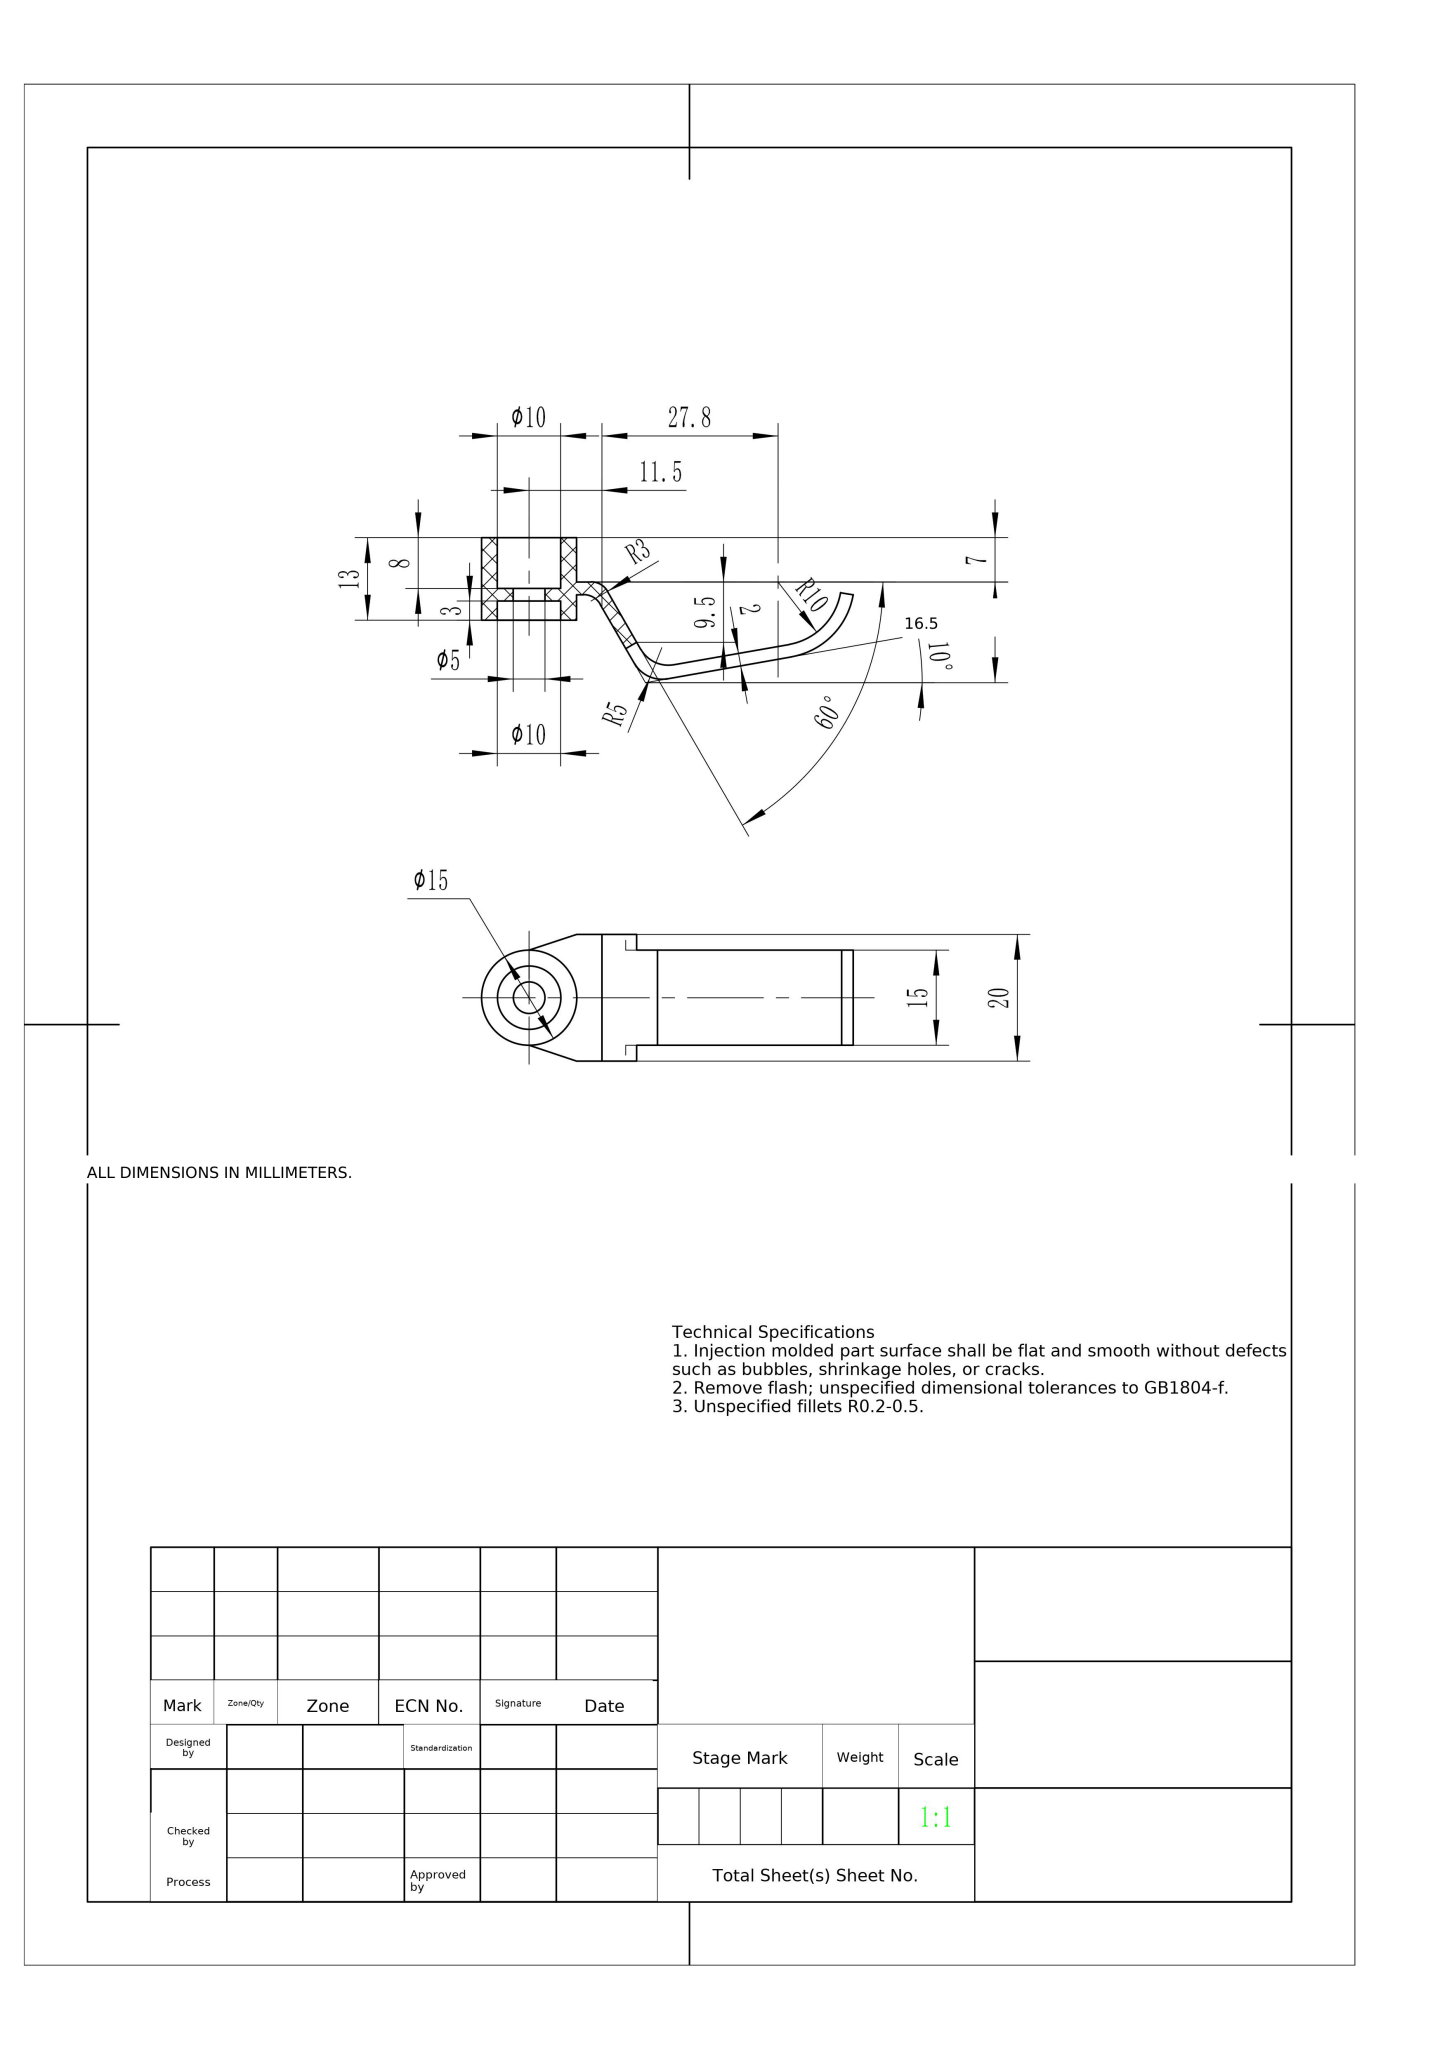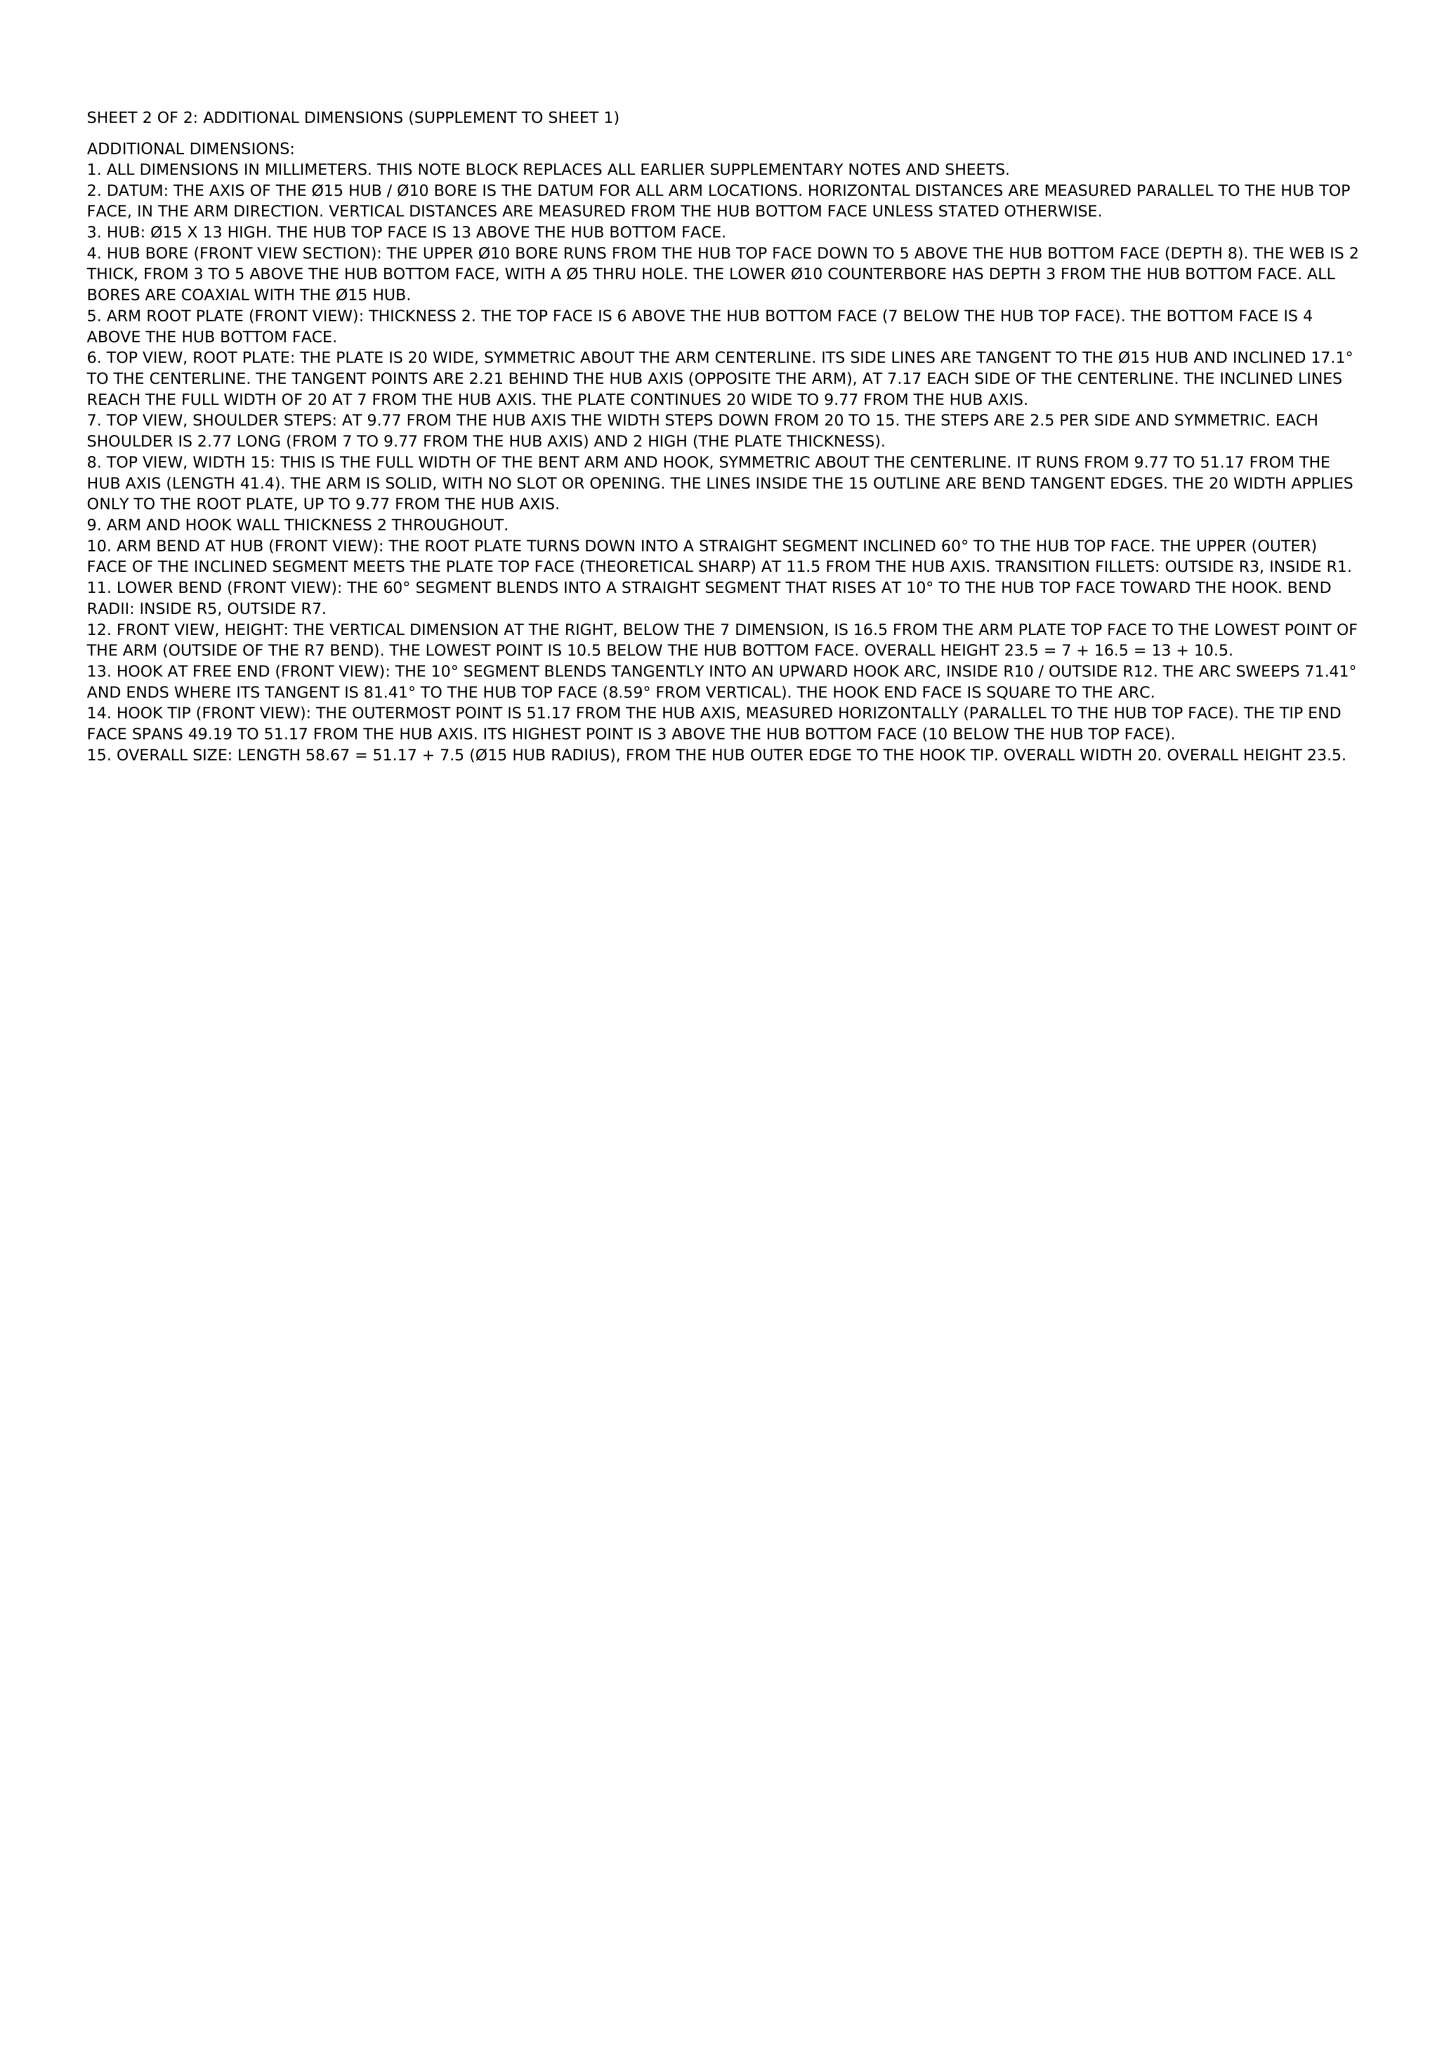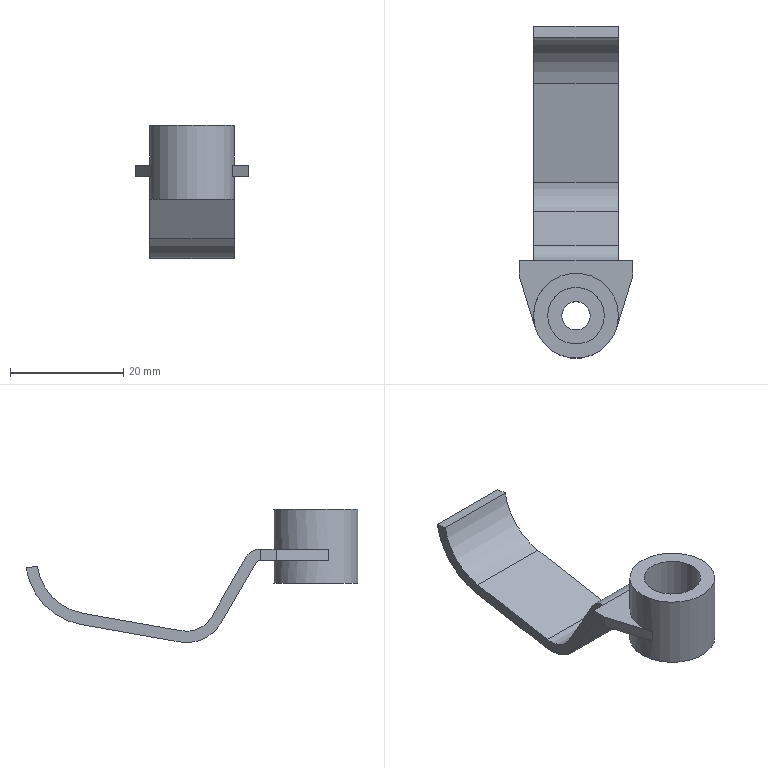Part | NX | mm | 1 solid | 29 faces | box 20 x 58.67 x 23.5 mm | volume 3167 mm3 | plane 19 | cylinder 10 | commonest cylinder face diameters 10 x3 2 x1 14 x1 24 x1 20 x1 6 x1 15 x1 5 x1
STEP:
#1=CARTESIAN_POINT('',(0.,0.,0.));
#2=DIRECTION('',(0.,0.,1.));
#3=DIRECTION('',(1.,0.,0.));
#4=AXIS2_PLACEMENT_3D('',#1,#2,#3);
#5=(LENGTH_UNIT()NAMED_UNIT(*)SI_UNIT(.MILLI.,.METRE.));
#6=UNCERTAINTY_MEASURE_WITH_UNIT(LENGTH_MEASURE(0.00002),#5,'','');
#7=(NAMED_UNIT(*)PLANE_ANGLE_UNIT()SI_UNIT($,.RADIAN.));
#8=PLANE_ANGLE_MEASURE_WITH_UNIT(PLANE_ANGLE_MEASURE(0.01745),#7);
#9=DIMENSIONAL_EXPONENTS(0.,0.,0.,0.,0.,0.,0.);
#10=(CONVERSION_BASED_UNIT('',#8)NAMED_UNIT(#9)PLANE_ANGLE_UNIT());
#11=(NAMED_UNIT(*)SI_UNIT($,.STERADIAN.)SOLID_ANGLE_UNIT());
#12=(GEOMETRIC_REPRESENTATION_CONTEXT(3)GLOBAL_UNCERTAINTY_ASSIGNED_CONTEXT((#6))GLOBAL_UNIT_ASSIGNED_CONTEXT((#5,#10,#11))REPRESENTATION_CONTEXT('',''));
#13=SHAPE_REPRESENTATION('',(#4),#12);
#14=CARTESIAN_POINT('',(10.,9.768,6.));
#15=VERTEX_POINT('',#14);
#16=CARTESIAN_POINT('',(10.,9.768,4.));
#17=VERTEX_POINT('',#16);
#18=CARTESIAN_POINT('',(10.,9.768,8.));
#19=DIRECTION('',(0.,0.,-1.));
#20=VECTOR('',#19,1.);
#21=LINE('',#18,#20);
#22=EDGE_CURVE('',#15,#17,#21,.T.);
#23=ORIENTED_EDGE('',*,*,#22,.F.);
#24=CARTESIAN_POINT('',(10.,7.,6.));
#25=VERTEX_POINT('',#24);
#26=CARTESIAN_POINT('',(10.,9.768,6.));
#27=DIRECTION('',(0.,-1.,-0.));
#28=VECTOR('',#27,1.);
#29=LINE('',#26,#28);
#30=EDGE_CURVE('',#15,#25,#29,.T.);
#31=ORIENTED_EDGE('',*,*,#30,.T.);
#32=CARTESIAN_POINT('',(10.,7.,4.));
#33=VERTEX_POINT('',#32);
#34=CARTESIAN_POINT('',(10.,7.,6.));
#35=DIRECTION('',(0.,0.,-1.));
#36=VECTOR('',#35,1.);
#37=LINE('',#34,#36);
#38=EDGE_CURVE('',#25,#33,#37,.T.);
#39=ORIENTED_EDGE('',*,*,#38,.T.);
#40=CARTESIAN_POINT('',(10.,7.,4.));
#41=DIRECTION('',(0.,1.,0.));
#42=VECTOR('',#41,1.);
#43=LINE('',#40,#42);
#44=EDGE_CURVE('',#33,#17,#43,.T.);
#45=ORIENTED_EDGE('',*,*,#44,.T.);
#46=EDGE_LOOP('',(#23,#31,#39,#45));
#47=FACE_OUTER_BOUND('',#46,.T.);
#48=CARTESIAN_POINT('',(10.,9.768,3.));
#49=DIRECTION('',(-1.,0.,0.));
#50=DIRECTION('',(0.,0.,1.));
#51=AXIS2_PLACEMENT_3D('',#48,#49,#50);
#52=PLANE('',#51);
#53=ADVANCED_FACE('',(#47),#52,.F.);
#54=CARTESIAN_POINT('',(7.5,10.634,3.5));
#55=VERTEX_POINT('',#54);
#56=CARTESIAN_POINT('',(-7.5,10.634,3.5));
#57=VERTEX_POINT('',#56);
#58=CARTESIAN_POINT('',(10.,10.634,3.5));
#59=DIRECTION('',(-1.,0.,0.));
#60=VECTOR('',#59,1.);
#61=LINE('',#58,#60);
#62=EDGE_CURVE('',#55,#57,#61,.T.);
#63=ORIENTED_EDGE('',*,*,#62,.F.);
#64=CARTESIAN_POINT('',(7.5,9.768,4.));
#65=VERTEX_POINT('',#64);
#66=CARTESIAN_POINT('',(7.5,9.768,3.));
#67=DIRECTION('',(1.,-0.,-0.));
#68=DIRECTION('',(0.,-1.,0.));
#69=AXIS2_PLACEMENT_3D('',#66,#67,#68);
#70=CIRCLE('',#69,1.);
#71=EDGE_CURVE('',#55,#65,#70,.T.);
#72=ORIENTED_EDGE('',*,*,#71,.T.);
#73=CARTESIAN_POINT('',(-7.5,9.768,4.));
#74=VERTEX_POINT('',#73);
#75=CARTESIAN_POINT('',(10.,9.768,4.));
#76=DIRECTION('',(-1.,0.,0.));
#77=VECTOR('',#76,1.);
#78=LINE('',#75,#77);
#79=EDGE_CURVE('',#65,#74,#78,.T.);
#80=ORIENTED_EDGE('',*,*,#79,.T.);
#81=CARTESIAN_POINT('',(-7.5,9.768,3.));
#82=DIRECTION('',(1.,0.,0.));
#83=DIRECTION('',(0.,-1.,0.));
#84=AXIS2_PLACEMENT_3D('',#81,#82,#83);
#85=CIRCLE('',#84,1.);
#86=EDGE_CURVE('',#57,#74,#85,.T.);
#87=ORIENTED_EDGE('',*,*,#86,.F.);
#88=EDGE_LOOP('',(#63,#72,#80,#87));
#89=FACE_OUTER_BOUND('',#88,.T.);
#90=CARTESIAN_POINT('',(10.,9.768,3.));
#91=DIRECTION('',(-1.,0.,0.));
#92=DIRECTION('',(0.,0.,1.));
#93=AXIS2_PLACEMENT_3D('',#90,#91,#92);
#94=CYLINDRICAL_SURFACE('',#93,1.);
#95=ADVANCED_FACE('',(#89),#94,.F.);
#96=CARTESIAN_POINT('',(7.5,16.696,-7.));
#97=VERTEX_POINT('',#96);
#98=CARTESIAN_POINT('',(-7.5,16.696,-7.));
#99=VERTEX_POINT('',#98);
#100=CARTESIAN_POINT('',(10.,16.696,-7.));
#101=DIRECTION('',(-1.,0.,0.));
#102=VECTOR('',#101,1.);
#103=LINE('',#100,#102);
#104=EDGE_CURVE('',#97,#99,#103,.T.);
#105=ORIENTED_EDGE('',*,*,#104,.F.);
#106=CARTESIAN_POINT('',(7.5,10.634,3.5));
#107=DIRECTION('',(-0.,-0.5,0.866));
#108=VECTOR('',#107,1.);
#109=LINE('',#106,#108);
#110=EDGE_CURVE('',#97,#55,#109,.T.);
#111=ORIENTED_EDGE('',*,*,#110,.T.);
#112=ORIENTED_EDGE('',*,*,#62,.T.);
#113=CARTESIAN_POINT('',(-7.5,10.634,3.5));
#114=DIRECTION('',(0.,-0.5,0.866));
#115=VECTOR('',#114,1.);
#116=LINE('',#113,#115);
#117=EDGE_CURVE('',#99,#57,#116,.T.);
#118=ORIENTED_EDGE('',*,*,#117,.F.);
#119=EDGE_LOOP('',(#105,#111,#112,#118));
#120=FACE_OUTER_BOUND('',#119,.T.);
#121=CARTESIAN_POINT('',(10.,10.634,3.5));
#122=DIRECTION('',(0.,0.866,0.5));
#123=DIRECTION('',(0.,-0.5,0.866));
#124=AXIS2_PLACEMENT_3D('',#121,#122,#123);
#125=PLANE('',#124);
#126=ADVANCED_FACE('',(#120),#125,.F.);
#127=CARTESIAN_POINT('',(7.5,23.974,-10.394));
#128=VERTEX_POINT('',#127);
#129=CARTESIAN_POINT('',(-7.5,23.974,-10.394));
#130=VERTEX_POINT('',#129);
#131=CARTESIAN_POINT('',(10.,23.974,-10.394));
#132=DIRECTION('',(-1.,0.,0.));
#133=VECTOR('',#132,1.);
#134=LINE('',#131,#133);
#135=EDGE_CURVE('',#128,#130,#134,.T.);
#136=ORIENTED_EDGE('',*,*,#135,.F.);
#137=CARTESIAN_POINT('',(7.5,22.758,-3.5));
#138=DIRECTION('',(-1.,0.,0.));
#139=DIRECTION('',(-0.,-1.,0.));
#140=AXIS2_PLACEMENT_3D('',#137,#138,#139);
#141=CIRCLE('',#140,7.);
#142=EDGE_CURVE('',#128,#97,#141,.T.);
#143=ORIENTED_EDGE('',*,*,#142,.T.);
#144=ORIENTED_EDGE('',*,*,#104,.T.);
#145=CARTESIAN_POINT('',(-7.5,22.758,-3.5));
#146=DIRECTION('',(-1.,-0.,-0.));
#147=DIRECTION('',(0.,-1.,0.));
#148=AXIS2_PLACEMENT_3D('',#145,#146,#147);
#149=CIRCLE('',#148,7.);
#150=EDGE_CURVE('',#130,#99,#149,.T.);
#151=ORIENTED_EDGE('',*,*,#150,.F.);
#152=EDGE_LOOP('',(#136,#143,#144,#151));
#153=FACE_OUTER_BOUND('',#152,.T.);
#154=CARTESIAN_POINT('',(10.,22.758,-3.5));
#155=DIRECTION('',(-1.,0.,0.));
#156=DIRECTION('',(0.,0.,1.));
#157=AXIS2_PLACEMENT_3D('',#154,#155,#156);
#158=CYLINDRICAL_SURFACE('',#157,7.);
#159=ADVANCED_FACE('',(#153),#158,.T.);
#160=CARTESIAN_POINT('',(7.5,41.384,-7.324));
#161=VERTEX_POINT('',#160);
#162=CARTESIAN_POINT('',(-7.5,41.384,-7.324));
#163=VERTEX_POINT('',#162);
#164=CARTESIAN_POINT('',(10.,41.384,-7.324));
#165=DIRECTION('',(-1.,0.,0.));
#166=VECTOR('',#165,1.);
#167=LINE('',#164,#166);
#168=EDGE_CURVE('',#161,#163,#167,.T.);
#169=ORIENTED_EDGE('',*,*,#168,.F.);
#170=CARTESIAN_POINT('',(7.5,23.974,-10.394));
#171=DIRECTION('',(-0.,-0.9848,-0.1736));
#172=VECTOR('',#171,1.);
#173=LINE('',#170,#172);
#174=EDGE_CURVE('',#161,#128,#173,.T.);
#175=ORIENTED_EDGE('',*,*,#174,.T.);
#176=ORIENTED_EDGE('',*,*,#135,.T.);
#177=CARTESIAN_POINT('',(-7.5,23.974,-10.394));
#178=DIRECTION('',(0.,-0.9848,-0.1736));
#179=VECTOR('',#178,1.);
#180=LINE('',#177,#179);
#181=EDGE_CURVE('',#163,#130,#180,.T.);
#182=ORIENTED_EDGE('',*,*,#181,.F.);
#183=EDGE_LOOP('',(#169,#175,#176,#182));
#184=FACE_OUTER_BOUND('',#183,.T.);
#185=CARTESIAN_POINT('',(10.,23.974,-10.394));
#186=DIRECTION('',(0.,-0.1736,0.9848));
#187=DIRECTION('',(0.,-0.9848,-0.1736));
#188=AXIS2_PLACEMENT_3D('',#185,#186,#187);
#189=PLANE('',#188);
#190=ADVANCED_FACE('',(#184),#189,.F.);
#191=CARTESIAN_POINT('',(7.5,51.165,2.701));
#192=VERTEX_POINT('',#191);
#193=CARTESIAN_POINT('',(-7.5,51.165,2.701));
#194=VERTEX_POINT('',#193);
#195=CARTESIAN_POINT('',(10.,51.165,2.701));
#196=DIRECTION('',(-1.,0.,0.));
#197=VECTOR('',#196,1.);
#198=LINE('',#195,#197);
#199=EDGE_CURVE('',#192,#194,#198,.T.);
#200=ORIENTED_EDGE('',*,*,#199,.F.);
#201=CARTESIAN_POINT('',(7.5,39.3,4.494));
#202=DIRECTION('',(-1.,0.,0.));
#203=DIRECTION('',(-0.,-1.,0.));
#204=AXIS2_PLACEMENT_3D('',#201,#202,#203);
#205=CIRCLE('',#204,12.);
#206=EDGE_CURVE('',#192,#161,#205,.T.);
#207=ORIENTED_EDGE('',*,*,#206,.T.);
#208=ORIENTED_EDGE('',*,*,#168,.T.);
#209=CARTESIAN_POINT('',(-7.5,39.3,4.494));
#210=DIRECTION('',(-1.,-0.,-0.));
#211=DIRECTION('',(0.,-1.,0.));
#212=AXIS2_PLACEMENT_3D('',#209,#210,#211);
#213=CIRCLE('',#212,12.);
#214=EDGE_CURVE('',#194,#163,#213,.T.);
#215=ORIENTED_EDGE('',*,*,#214,.F.);
#216=EDGE_LOOP('',(#200,#207,#208,#215));
#217=FACE_OUTER_BOUND('',#216,.T.);
#218=CARTESIAN_POINT('',(10.,39.3,4.494));
#219=DIRECTION('',(-1.,0.,0.));
#220=DIRECTION('',(0.,0.,1.));
#221=AXIS2_PLACEMENT_3D('',#218,#219,#220);
#222=CYLINDRICAL_SURFACE('',#221,12.);
#223=ADVANCED_FACE('',(#217),#222,.T.);
#224=CARTESIAN_POINT('',(7.5,49.188,3.));
#225=VERTEX_POINT('',#224);
#226=CARTESIAN_POINT('',(-7.5,49.188,3.));
#227=VERTEX_POINT('',#226);
#228=CARTESIAN_POINT('',(10.,49.188,3.));
#229=DIRECTION('',(-1.,0.,0.));
#230=VECTOR('',#229,1.);
#231=LINE('',#228,#230);
#232=EDGE_CURVE('',#225,#227,#231,.T.);
#233=ORIENTED_EDGE('',*,*,#232,.F.);
#234=CARTESIAN_POINT('',(7.5,51.165,2.701));
#235=DIRECTION('',(0.,0.9888,-0.1494));
#236=VECTOR('',#235,1.);
#237=LINE('',#234,#236);
#238=EDGE_CURVE('',#225,#192,#237,.T.);
#239=ORIENTED_EDGE('',*,*,#238,.T.);
#240=ORIENTED_EDGE('',*,*,#199,.T.);
#241=CARTESIAN_POINT('',(-7.5,51.165,2.701));
#242=DIRECTION('',(-0.,0.9888,-0.1494));
#243=VECTOR('',#242,1.);
#244=LINE('',#241,#243);
#245=EDGE_CURVE('',#227,#194,#244,.T.);
#246=ORIENTED_EDGE('',*,*,#245,.F.);
#247=EDGE_LOOP('',(#233,#239,#240,#246));
#248=FACE_OUTER_BOUND('',#247,.T.);
#249=CARTESIAN_POINT('',(10.,51.165,2.701));
#250=DIRECTION('',(0.,-0.1494,-0.9888));
#251=DIRECTION('',(0.,0.9888,-0.1494));
#252=AXIS2_PLACEMENT_3D('',#249,#250,#251);
#253=PLANE('',#252);
#254=ADVANCED_FACE('',(#248),#253,.F.);
#255=CARTESIAN_POINT('',(7.5,41.036,-5.354));
#256=VERTEX_POINT('',#255);
#257=CARTESIAN_POINT('',(-7.5,41.036,-5.354));
#258=VERTEX_POINT('',#257);
#259=CARTESIAN_POINT('',(10.,41.036,-5.354));
#260=DIRECTION('',(-1.,0.,0.));
#261=VECTOR('',#260,1.);
#262=LINE('',#259,#261);
#263=EDGE_CURVE('',#256,#258,#262,.T.);
#264=ORIENTED_EDGE('',*,*,#263,.F.);
#265=CARTESIAN_POINT('',(7.5,39.3,4.494));
#266=DIRECTION('',(1.,-0.,-0.));
#267=DIRECTION('',(-0.,-1.,0.));
#268=AXIS2_PLACEMENT_3D('',#265,#266,#267);
#269=CIRCLE('',#268,10.);
#270=EDGE_CURVE('',#256,#225,#269,.T.);
#271=ORIENTED_EDGE('',*,*,#270,.T.);
#272=ORIENTED_EDGE('',*,*,#232,.T.);
#273=CARTESIAN_POINT('',(-7.5,39.3,4.494));
#274=DIRECTION('',(1.,0.,0.));
#275=DIRECTION('',(0.,-1.,0.));
#276=AXIS2_PLACEMENT_3D('',#273,#274,#275);
#277=CIRCLE('',#276,10.);
#278=EDGE_CURVE('',#258,#227,#277,.T.);
#279=ORIENTED_EDGE('',*,*,#278,.F.);
#280=EDGE_LOOP('',(#264,#271,#272,#279));
#281=FACE_OUTER_BOUND('',#280,.T.);
#282=CARTESIAN_POINT('',(10.,39.3,4.494));
#283=DIRECTION('',(-1.,0.,0.));
#284=DIRECTION('',(0.,0.,1.));
#285=AXIS2_PLACEMENT_3D('',#282,#283,#284);
#286=CYLINDRICAL_SURFACE('',#285,10.);
#287=ADVANCED_FACE('',(#281),#286,.F.);
#288=CARTESIAN_POINT('',(7.5,23.627,-8.424));
#289=VERTEX_POINT('',#288);
#290=CARTESIAN_POINT('',(-7.5,23.627,-8.424));
#291=VERTEX_POINT('',#290);
#292=CARTESIAN_POINT('',(10.,23.627,-8.424));
#293=DIRECTION('',(-1.,0.,0.));
#294=VECTOR('',#293,1.);
#295=LINE('',#292,#294);
#296=EDGE_CURVE('',#289,#291,#295,.T.);
#297=ORIENTED_EDGE('',*,*,#296,.F.);
#298=CARTESIAN_POINT('',(7.5,41.036,-5.354));
#299=DIRECTION('',(0.,0.9848,0.1736));
#300=VECTOR('',#299,1.);
#301=LINE('',#298,#300);
#302=EDGE_CURVE('',#289,#256,#301,.T.);
#303=ORIENTED_EDGE('',*,*,#302,.T.);
#304=ORIENTED_EDGE('',*,*,#263,.T.);
#305=CARTESIAN_POINT('',(-7.5,41.036,-5.354));
#306=DIRECTION('',(-0.,0.9848,0.1736));
#307=VECTOR('',#306,1.);
#308=LINE('',#305,#307);
#309=EDGE_CURVE('',#291,#258,#308,.T.);
#310=ORIENTED_EDGE('',*,*,#309,.F.);
#311=EDGE_LOOP('',(#297,#303,#304,#310));
#312=FACE_OUTER_BOUND('',#311,.T.);
#313=CARTESIAN_POINT('',(10.,41.036,-5.354));
#314=DIRECTION('',(0.,0.1736,-0.9848));
#315=DIRECTION('',(0.,0.9848,0.1736));
#316=AXIS2_PLACEMENT_3D('',#313,#314,#315);
#317=PLANE('',#316);
#318=ADVANCED_FACE('',(#312),#317,.F.);
#319=CARTESIAN_POINT('',(7.5,18.428,-6.));
#320=VERTEX_POINT('',#319);
#321=CARTESIAN_POINT('',(-7.5,18.428,-6.));
#322=VERTEX_POINT('',#321);
#323=CARTESIAN_POINT('',(10.,18.428,-6.));
#324=DIRECTION('',(-1.,0.,0.));
#325=VECTOR('',#324,1.);
#326=LINE('',#323,#325);
#327=EDGE_CURVE('',#320,#322,#326,.T.);
#328=ORIENTED_EDGE('',*,*,#327,.F.);
#329=CARTESIAN_POINT('',(7.5,22.758,-3.5));
#330=DIRECTION('',(1.,-0.,-0.));
#331=DIRECTION('',(-0.,-1.,0.));
#332=AXIS2_PLACEMENT_3D('',#329,#330,#331);
#333=CIRCLE('',#332,5.);
#334=EDGE_CURVE('',#320,#289,#333,.T.);
#335=ORIENTED_EDGE('',*,*,#334,.T.);
#336=ORIENTED_EDGE('',*,*,#296,.T.);
#337=CARTESIAN_POINT('',(-7.5,22.758,-3.5));
#338=DIRECTION('',(1.,0.,0.));
#339=DIRECTION('',(0.,-1.,0.));
#340=AXIS2_PLACEMENT_3D('',#337,#338,#339);
#341=CIRCLE('',#340,5.);
#342=EDGE_CURVE('',#322,#291,#341,.T.);
#343=ORIENTED_EDGE('',*,*,#342,.F.);
#344=EDGE_LOOP('',(#328,#335,#336,#343));
#345=FACE_OUTER_BOUND('',#344,.T.);
#346=CARTESIAN_POINT('',(10.,22.758,-3.5));
#347=DIRECTION('',(-1.,0.,0.));
#348=DIRECTION('',(0.,0.,1.));
#349=AXIS2_PLACEMENT_3D('',#346,#347,#348);
#350=CYLINDRICAL_SURFACE('',#349,5.);
#351=ADVANCED_FACE('',(#345),#350,.F.);
#352=CARTESIAN_POINT('',(7.5,12.366,4.5));
#353=VERTEX_POINT('',#352);
#354=CARTESIAN_POINT('',(-7.5,12.366,4.5));
#355=VERTEX_POINT('',#354);
#356=CARTESIAN_POINT('',(10.,12.366,4.5));
#357=DIRECTION('',(-1.,0.,0.));
#358=VECTOR('',#357,1.);
#359=LINE('',#356,#358);
#360=EDGE_CURVE('',#353,#355,#359,.T.);
#361=ORIENTED_EDGE('',*,*,#360,.F.);
#362=CARTESIAN_POINT('',(7.5,18.428,-6.));
#363=DIRECTION('',(0.,0.5,-0.866));
#364=VECTOR('',#363,1.);
#365=LINE('',#362,#364);
#366=EDGE_CURVE('',#353,#320,#365,.T.);
#367=ORIENTED_EDGE('',*,*,#366,.T.);
#368=ORIENTED_EDGE('',*,*,#327,.T.);
#369=CARTESIAN_POINT('',(-7.5,18.428,-6.));
#370=DIRECTION('',(-0.,0.5,-0.866));
#371=VECTOR('',#370,1.);
#372=LINE('',#369,#371);
#373=EDGE_CURVE('',#355,#322,#372,.T.);
#374=ORIENTED_EDGE('',*,*,#373,.F.);
#375=EDGE_LOOP('',(#361,#367,#368,#374));
#376=FACE_OUTER_BOUND('',#375,.T.);
#377=CARTESIAN_POINT('',(10.,18.428,-6.));
#378=DIRECTION('',(0.,-0.866,-0.5));
#379=DIRECTION('',(0.,0.5,-0.866));
#380=AXIS2_PLACEMENT_3D('',#377,#378,#379);
#381=PLANE('',#380);
#382=ADVANCED_FACE('',(#376),#381,.F.);
#383=CARTESIAN_POINT('',(7.5,9.768,6.));
#384=VERTEX_POINT('',#383);
#385=CARTESIAN_POINT('',(-7.5,9.768,6.));
#386=VERTEX_POINT('',#385);
#387=CARTESIAN_POINT('',(10.,9.768,6.));
#388=DIRECTION('',(-1.,0.,0.));
#389=VECTOR('',#388,1.);
#390=LINE('',#387,#389);
#391=EDGE_CURVE('',#384,#386,#390,.T.);
#392=ORIENTED_EDGE('',*,*,#391,.F.);
#393=CARTESIAN_POINT('',(7.5,9.768,3.));
#394=DIRECTION('',(-1.,0.,0.));
#395=DIRECTION('',(0.,-1.,0.));
#396=AXIS2_PLACEMENT_3D('',#393,#394,#395);
#397=CIRCLE('',#396,3.);
#398=EDGE_CURVE('',#384,#353,#397,.T.);
#399=ORIENTED_EDGE('',*,*,#398,.T.);
#400=ORIENTED_EDGE('',*,*,#360,.T.);
#401=CARTESIAN_POINT('',(-7.5,9.768,3.));
#402=DIRECTION('',(-1.,-0.,-0.));
#403=DIRECTION('',(0.,-1.,0.));
#404=AXIS2_PLACEMENT_3D('',#401,#402,#403);
#405=CIRCLE('',#404,3.);
#406=EDGE_CURVE('',#386,#355,#405,.T.);
#407=ORIENTED_EDGE('',*,*,#406,.F.);
#408=EDGE_LOOP('',(#392,#399,#400,#407));
#409=FACE_OUTER_BOUND('',#408,.T.);
#410=CARTESIAN_POINT('',(10.,9.768,3.));
#411=DIRECTION('',(-1.,0.,0.));
#412=DIRECTION('',(0.,0.,1.));
#413=AXIS2_PLACEMENT_3D('',#410,#411,#412);
#414=CYLINDRICAL_SURFACE('',#413,3.);
#415=ADVANCED_FACE('',(#409),#414,.T.);
#416=CARTESIAN_POINT('',(-10.,9.768,6.));
#417=VERTEX_POINT('',#416);
#418=CARTESIAN_POINT('',(-10.,7.,6.));
#419=VERTEX_POINT('',#418);
#420=CARTESIAN_POINT('',(-10.,9.768,6.));
#421=DIRECTION('',(0.,-1.,-0.));
#422=VECTOR('',#421,1.);
#423=LINE('',#420,#422);
#424=EDGE_CURVE('',#417,#419,#423,.T.);
#425=ORIENTED_EDGE('',*,*,#424,.F.);
#426=CARTESIAN_POINT('',(-10.,9.768,4.));
#427=VERTEX_POINT('',#426);
#428=CARTESIAN_POINT('',(-10.,9.768,8.));
#429=DIRECTION('',(0.,0.,-1.));
#430=VECTOR('',#429,1.);
#431=LINE('',#428,#430);
#432=EDGE_CURVE('',#417,#427,#431,.T.);
#433=ORIENTED_EDGE('',*,*,#432,.T.);
#434=CARTESIAN_POINT('',(-10.,7.,4.));
#435=VERTEX_POINT('',#434);
#436=CARTESIAN_POINT('',(-10.,7.,4.));
#437=DIRECTION('',(0.,1.,0.));
#438=VECTOR('',#437,1.);
#439=LINE('',#436,#438);
#440=EDGE_CURVE('',#435,#427,#439,.T.);
#441=ORIENTED_EDGE('',*,*,#440,.F.);
#442=CARTESIAN_POINT('',(-10.,7.,6.));
#443=DIRECTION('',(0.,0.,-1.));
#444=VECTOR('',#443,1.);
#445=LINE('',#442,#444);
#446=EDGE_CURVE('',#419,#435,#445,.T.);
#447=ORIENTED_EDGE('',*,*,#446,.F.);
#448=EDGE_LOOP('',(#425,#433,#441,#447));
#449=FACE_OUTER_BOUND('',#448,.T.);
#450=CARTESIAN_POINT('',(-10.,9.768,3.));
#451=DIRECTION('',(-1.,0.,0.));
#452=DIRECTION('',(0.,0.,1.));
#453=AXIS2_PLACEMENT_3D('',#450,#451,#452);
#454=PLANE('',#453);
#455=ADVANCED_FACE('',(#449),#454,.T.);
#456=CARTESIAN_POINT('',(7.169,-2.205,4.));
#457=VERTEX_POINT('',#456);
#458=CARTESIAN_POINT('',(7.169,-2.205,6.));
#459=VERTEX_POINT('',#458);
#460=CARTESIAN_POINT('',(7.169,-2.205,4.));
#461=DIRECTION('',(0.,-0.,1.));
#462=VECTOR('',#461,1.);
#463=LINE('',#460,#462);
#464=EDGE_CURVE('',#457,#459,#463,.T.);
#465=ORIENTED_EDGE('',*,*,#464,.T.);
#466=CARTESIAN_POINT('',(-7.169,-2.205,6.));
#467=VERTEX_POINT('',#466);
#468=CARTESIAN_POINT('',(0.,0.,6.));
#469=DIRECTION('',(0.,0.,-1.));
#470=DIRECTION('',(0.,1.,0.));
#471=AXIS2_PLACEMENT_3D('',#468,#469,#470);
#472=CIRCLE('',#471,7.5);
#473=EDGE_CURVE('',#467,#459,#472,.T.);
#474=ORIENTED_EDGE('',*,*,#473,.F.);
#475=CARTESIAN_POINT('',(-7.169,-2.205,4.));
#476=VERTEX_POINT('',#475);
#477=CARTESIAN_POINT('',(-7.169,-2.205,4.));
#478=DIRECTION('',(0.,-0.,1.));
#479=VECTOR('',#478,1.);
#480=LINE('',#477,#479);
#481=EDGE_CURVE('',#476,#467,#480,.T.);
#482=ORIENTED_EDGE('',*,*,#481,.F.);
#483=CARTESIAN_POINT('',(0.,0.,4.));
#484=DIRECTION('',(0.,0.,1.));
#485=DIRECTION('',(1.,0.,0.));
#486=AXIS2_PLACEMENT_3D('',#483,#484,#485);
#487=CIRCLE('',#486,7.5);
#488=EDGE_CURVE('',#457,#476,#487,.T.);
#489=ORIENTED_EDGE('',*,*,#488,.F.);
#490=EDGE_LOOP('',(#465,#474,#482,#489));
#491=FACE_BOUND('',#490,.T.);
#492=CARTESIAN_POINT('',(7.5,0.,13.));
#493=VERTEX_POINT('',#492);
#494=CARTESIAN_POINT('',(0.,0.,13.));
#495=DIRECTION('',(0.,0.,1.));
#496=DIRECTION('',(1.,0.,0.));
#497=AXIS2_PLACEMENT_3D('',#494,#495,#496);
#498=CIRCLE('',#497,7.5);
#499=EDGE_CURVE('',#493,#493,#498,.T.);
#500=ORIENTED_EDGE('',*,*,#499,.F.);
#501=EDGE_LOOP('',(#500));
#502=FACE_BOUND('',#501,.T.);
#503=CARTESIAN_POINT('',(7.5,0.,0.));
#504=VERTEX_POINT('',#503);
#505=CARTESIAN_POINT('',(0.,0.,0.));
#506=DIRECTION('',(0.,0.,1.));
#507=DIRECTION('',(1.,0.,0.));
#508=AXIS2_PLACEMENT_3D('',#505,#506,#507);
#509=CIRCLE('',#508,7.5);
#510=EDGE_CURVE('',#504,#504,#509,.T.);
#511=ORIENTED_EDGE('',*,*,#510,.T.);
#512=EDGE_LOOP('',(#511));
#513=FACE_BOUND('',#512,.T.);
#514=CARTESIAN_POINT('',(0.,0.,13.));
#515=DIRECTION('',(0.,0.,-1.));
#516=DIRECTION('',(-1.,0.,0.));
#517=AXIS2_PLACEMENT_3D('',#514,#515,#516);
#518=CYLINDRICAL_SURFACE('',#517,7.5);
#519=ADVANCED_FACE('',(#491,#502,#513),#518,.T.);
#520=CARTESIAN_POINT('',(2.5,0.,3.));
#521=VERTEX_POINT('',#520);
#522=CARTESIAN_POINT('',(0.,0.,3.));
#523=DIRECTION('',(0.,0.,1.));
#524=DIRECTION('',(1.,0.,0.));
#525=AXIS2_PLACEMENT_3D('',#522,#523,#524);
#526=CIRCLE('',#525,2.5);
#527=EDGE_CURVE('',#521,#521,#526,.T.);
#528=ORIENTED_EDGE('',*,*,#527,.F.);
#529=EDGE_LOOP('',(#528));
#530=FACE_BOUND('',#529,.T.);
#531=CARTESIAN_POINT('',(2.5,0.,5.));
#532=VERTEX_POINT('',#531);
#533=CARTESIAN_POINT('',(0.,0.,5.));
#534=DIRECTION('',(0.,0.,1.));
#535=DIRECTION('',(1.,0.,0.));
#536=AXIS2_PLACEMENT_3D('',#533,#534,#535);
#537=CIRCLE('',#536,2.5);
#538=EDGE_CURVE('',#532,#532,#537,.T.);
#539=ORIENTED_EDGE('',*,*,#538,.T.);
#540=EDGE_LOOP('',(#539));
#541=FACE_BOUND('',#540,.T.);
#542=CARTESIAN_POINT('',(0.,0.,13.));
#543=DIRECTION('',(0.,0.,-1.));
#544=DIRECTION('',(-1.,0.,0.));
#545=AXIS2_PLACEMENT_3D('',#542,#543,#544);
#546=CYLINDRICAL_SURFACE('',#545,2.5);
#547=ADVANCED_FACE('',(#530,#541),#546,.F.);
#548=CARTESIAN_POINT('',(5.,0.,13.));
#549=VERTEX_POINT('',#548);
#550=CARTESIAN_POINT('',(0.,0.,13.));
#551=DIRECTION('',(0.,0.,1.));
#552=DIRECTION('',(1.,0.,0.));
#553=AXIS2_PLACEMENT_3D('',#550,#551,#552);
#554=CIRCLE('',#553,5.);
#555=EDGE_CURVE('',#549,#549,#554,.T.);
#556=ORIENTED_EDGE('',*,*,#555,.F.);
#557=EDGE_LOOP('',(#556));
#558=FACE_BOUND('',#557,.T.);
#559=ORIENTED_EDGE('',*,*,#499,.T.);
#560=EDGE_LOOP('',(#559));
#561=FACE_BOUND('',#560,.T.);
#562=CARTESIAN_POINT('',(0.,0.,13.));
#563=DIRECTION('',(0.,0.,1.));
#564=DIRECTION('',(1.,0.,0.));
#565=AXIS2_PLACEMENT_3D('',#562,#563,#564);
#566=PLANE('',#565);
#567=ADVANCED_FACE('',(#558,#561),#566,.T.);
#568=CARTESIAN_POINT('',(5.,0.,0.));
#569=VERTEX_POINT('',#568);
#570=CARTESIAN_POINT('',(0.,0.,0.));
#571=DIRECTION('',(0.,0.,1.));
#572=DIRECTION('',(1.,0.,0.));
#573=AXIS2_PLACEMENT_3D('',#570,#571,#572);
#574=CIRCLE('',#573,5.);
#575=EDGE_CURVE('',#569,#569,#574,.T.);
#576=ORIENTED_EDGE('',*,*,#575,.T.);
#577=EDGE_LOOP('',(#576));
#578=FACE_BOUND('',#577,.T.);
#579=ORIENTED_EDGE('',*,*,#510,.F.);
#580=EDGE_LOOP('',(#579));
#581=FACE_BOUND('',#580,.T.);
#582=CARTESIAN_POINT('',(0.,0.,0.));
#583=DIRECTION('',(0.,0.,1.));
#584=DIRECTION('',(1.,0.,0.));
#585=AXIS2_PLACEMENT_3D('',#582,#583,#584);
#586=PLANE('',#585);
#587=ADVANCED_FACE('',(#578,#581),#586,.F.);
#588=CARTESIAN_POINT('',(5.,0.,5.));
#589=VERTEX_POINT('',#588);
#590=CARTESIAN_POINT('',(0.,0.,5.));
#591=DIRECTION('',(0.,0.,-1.));
#592=DIRECTION('',(1.,0.,0.));
#593=AXIS2_PLACEMENT_3D('',#590,#591,#592);
#594=CIRCLE('',#593,5.);
#595=EDGE_CURVE('',#589,#589,#594,.T.);
#596=ORIENTED_EDGE('',*,*,#595,.T.);
#597=EDGE_LOOP('',(#596));
#598=FACE_BOUND('',#597,.T.);
#599=ORIENTED_EDGE('',*,*,#555,.T.);
#600=EDGE_LOOP('',(#599));
#601=FACE_BOUND('',#600,.T.);
#602=CARTESIAN_POINT('',(0.,0.,5.));
#603=DIRECTION('',(0.,0.,1.));
#604=DIRECTION('',(1.,0.,0.));
#605=AXIS2_PLACEMENT_3D('',#602,#603,#604);
#606=CYLINDRICAL_SURFACE('',#605,5.);
#607=ADVANCED_FACE('',(#598,#601),#606,.F.);
#608=ORIENTED_EDGE('',*,*,#538,.F.);
#609=EDGE_LOOP('',(#608));
#610=FACE_BOUND('',#609,.T.);
#611=ORIENTED_EDGE('',*,*,#595,.F.);
#612=EDGE_LOOP('',(#611));
#613=FACE_BOUND('',#612,.T.);
#614=CARTESIAN_POINT('',(0.,0.,5.));
#615=DIRECTION('',(0.,0.,1.));
#616=DIRECTION('',(1.,0.,0.));
#617=AXIS2_PLACEMENT_3D('',#614,#615,#616);
#618=PLANE('',#617);
#619=ADVANCED_FACE('',(#610,#613),#618,.T.);
#620=CARTESIAN_POINT('',(5.,0.,3.));
#621=VERTEX_POINT('',#620);
#622=CARTESIAN_POINT('',(0.,0.,3.));
#623=DIRECTION('',(0.,0.,-1.));
#624=DIRECTION('',(1.,0.,0.));
#625=AXIS2_PLACEMENT_3D('',#622,#623,#624);
#626=CIRCLE('',#625,5.);
#627=EDGE_CURVE('',#621,#621,#626,.T.);
#628=ORIENTED_EDGE('',*,*,#627,.F.);
#629=EDGE_LOOP('',(#628));
#630=FACE_BOUND('',#629,.T.);
#631=ORIENTED_EDGE('',*,*,#575,.F.);
#632=EDGE_LOOP('',(#631));
#633=FACE_BOUND('',#632,.T.);
#634=CARTESIAN_POINT('',(0.,0.,3.));
#635=DIRECTION('',(0.,0.,-1.));
#636=DIRECTION('',(-1.,0.,0.));
#637=AXIS2_PLACEMENT_3D('',#634,#635,#636);
#638=CYLINDRICAL_SURFACE('',#637,5.);
#639=ADVANCED_FACE('',(#630,#633),#638,.F.);
#640=ORIENTED_EDGE('',*,*,#527,.T.);
#641=EDGE_LOOP('',(#640));
#642=FACE_BOUND('',#641,.T.);
#643=ORIENTED_EDGE('',*,*,#627,.T.);
#644=EDGE_LOOP('',(#643));
#645=FACE_BOUND('',#644,.T.);
#646=CARTESIAN_POINT('',(0.,0.,3.));
#647=DIRECTION('',(0.,0.,1.));
#648=DIRECTION('',(1.,0.,0.));
#649=AXIS2_PLACEMENT_3D('',#646,#647,#648);
#650=PLANE('',#649);
#651=ADVANCED_FACE('',(#642,#645),#650,.F.);
#652=ORIENTED_EDGE('',*,*,#44,.F.);
#653=CARTESIAN_POINT('',(10.,7.,4.));
#654=DIRECTION('',(-0.294,-0.9558,-0.));
#655=VECTOR('',#654,1.);
#656=LINE('',#653,#655);
#657=EDGE_CURVE('',#33,#457,#656,.T.);
#658=ORIENTED_EDGE('',*,*,#657,.T.);
#659=ORIENTED_EDGE('',*,*,#488,.T.);
#660=CARTESIAN_POINT('',(-10.,7.,4.));
#661=DIRECTION('',(0.294,-0.9558,-0.));
#662=VECTOR('',#661,1.);
#663=LINE('',#660,#662);
#664=EDGE_CURVE('',#435,#476,#663,.T.);
#665=ORIENTED_EDGE('',*,*,#664,.F.);
#666=ORIENTED_EDGE('',*,*,#440,.T.);
#667=CARTESIAN_POINT('',(10.,9.768,4.));
#668=DIRECTION('',(-1.,0.,0.));
#669=VECTOR('',#668,1.);
#670=LINE('',#667,#669);
#671=EDGE_CURVE('',#74,#427,#670,.T.);
#672=ORIENTED_EDGE('',*,*,#671,.F.);
#673=ORIENTED_EDGE('',*,*,#79,.F.);
#674=CARTESIAN_POINT('',(10.,9.768,4.));
#675=DIRECTION('',(-1.,0.,0.));
#676=VECTOR('',#675,1.);
#677=LINE('',#674,#676);
#678=EDGE_CURVE('',#17,#65,#677,.T.);
#679=ORIENTED_EDGE('',*,*,#678,.F.);
#680=EDGE_LOOP('',(#652,#658,#659,#665,#666,#672,#673,#679));
#681=FACE_OUTER_BOUND('',#680,.T.);
#682=CARTESIAN_POINT('',(10.,7.,4.));
#683=DIRECTION('',(0.,0.,1.));
#684=DIRECTION('',(1.,0.,0.));
#685=AXIS2_PLACEMENT_3D('',#682,#683,#684);
#686=PLANE('',#685);
#687=ADVANCED_FACE('',(#681),#686,.F.);
#688=ORIENTED_EDGE('',*,*,#424,.T.);
#689=CARTESIAN_POINT('',(-10.,7.,6.));
#690=DIRECTION('',(0.294,-0.9558,-0.));
#691=VECTOR('',#690,1.);
#692=LINE('',#689,#691);
#693=EDGE_CURVE('',#419,#467,#692,.T.);
#694=ORIENTED_EDGE('',*,*,#693,.T.);
#695=ORIENTED_EDGE('',*,*,#473,.T.);
#696=CARTESIAN_POINT('',(10.,7.,6.));
#697=DIRECTION('',(-0.294,-0.9558,-0.));
#698=VECTOR('',#697,1.);
#699=LINE('',#696,#698);
#700=EDGE_CURVE('',#25,#459,#699,.T.);
#701=ORIENTED_EDGE('',*,*,#700,.F.);
#702=ORIENTED_EDGE('',*,*,#30,.F.);
#703=CARTESIAN_POINT('',(10.,9.768,6.));
#704=DIRECTION('',(-1.,0.,0.));
#705=VECTOR('',#704,1.);
#706=LINE('',#703,#705);
#707=EDGE_CURVE('',#15,#384,#706,.T.);
#708=ORIENTED_EDGE('',*,*,#707,.T.);
#709=ORIENTED_EDGE('',*,*,#391,.T.);
#710=CARTESIAN_POINT('',(10.,9.768,6.));
#711=DIRECTION('',(1.,-0.,-0.));
#712=VECTOR('',#711,1.);
#713=LINE('',#710,#712);
#714=EDGE_CURVE('',#417,#386,#713,.T.);
#715=ORIENTED_EDGE('',*,*,#714,.F.);
#716=EDGE_LOOP('',(#688,#694,#695,#701,#702,#708,#709,#715));
#717=FACE_OUTER_BOUND('',#716,.T.);
#718=CARTESIAN_POINT('',(10.,9.768,6.));
#719=DIRECTION('',(0.,0.,-1.));
#720=DIRECTION('',(0.,1.,0.));
#721=AXIS2_PLACEMENT_3D('',#718,#719,#720);
#722=PLANE('',#721);
#723=ADVANCED_FACE('',(#717),#722,.F.);
#724=ORIENTED_EDGE('',*,*,#693,.F.);
#725=ORIENTED_EDGE('',*,*,#446,.T.);
#726=ORIENTED_EDGE('',*,*,#664,.T.);
#727=ORIENTED_EDGE('',*,*,#481,.T.);
#728=EDGE_LOOP('',(#724,#725,#726,#727));
#729=FACE_OUTER_BOUND('',#728,.T.);
#730=CARTESIAN_POINT('',(-10.,7.,4.));
#731=DIRECTION('',(-0.9558,-0.294,-0.));
#732=DIRECTION('',(0.294,-0.9558,0.));
#733=AXIS2_PLACEMENT_3D('',#730,#731,#732);
#734=PLANE('',#733);
#735=ADVANCED_FACE('',(#729),#734,.T.);
#736=ORIENTED_EDGE('',*,*,#700,.T.);
#737=ORIENTED_EDGE('',*,*,#464,.F.);
#738=ORIENTED_EDGE('',*,*,#657,.F.);
#739=ORIENTED_EDGE('',*,*,#38,.F.);
#740=EDGE_LOOP('',(#736,#737,#738,#739));
#741=FACE_OUTER_BOUND('',#740,.T.);
#742=CARTESIAN_POINT('',(10.,7.,4.));
#743=DIRECTION('',(-0.9558,0.294,0.));
#744=DIRECTION('',(-0.294,-0.9558,0.));
#745=AXIS2_PLACEMENT_3D('',#742,#743,#744);
#746=PLANE('',#745);
#747=ADVANCED_FACE('',(#741),#746,.F.);
#748=ORIENTED_EDGE('',*,*,#86,.T.);
#749=CARTESIAN_POINT('',(-7.5,9.768,8.));
#750=DIRECTION('',(0.,-0.,1.));
#751=VECTOR('',#750,1.);
#752=LINE('',#749,#751);
#753=EDGE_CURVE('',#74,#386,#752,.T.);
#754=ORIENTED_EDGE('',*,*,#753,.T.);
#755=ORIENTED_EDGE('',*,*,#406,.T.);
#756=ORIENTED_EDGE('',*,*,#373,.T.);
#757=ORIENTED_EDGE('',*,*,#342,.T.);
#758=ORIENTED_EDGE('',*,*,#309,.T.);
#759=ORIENTED_EDGE('',*,*,#278,.T.);
#760=ORIENTED_EDGE('',*,*,#245,.T.);
#761=ORIENTED_EDGE('',*,*,#214,.T.);
#762=ORIENTED_EDGE('',*,*,#181,.T.);
#763=ORIENTED_EDGE('',*,*,#150,.T.);
#764=ORIENTED_EDGE('',*,*,#117,.T.);
#765=EDGE_LOOP('',(#748,#754,#755,#756,#757,#758,#759,#760,#761,#762,#763,#764));
#766=FACE_OUTER_BOUND('',#765,.T.);
#767=CARTESIAN_POINT('',(-7.5,9.768,8.));
#768=DIRECTION('',(-1.,-0.,-0.));
#769=DIRECTION('',(0.,-1.,0.));
#770=AXIS2_PLACEMENT_3D('',#767,#768,#769);
#771=PLANE('',#770);
#772=ADVANCED_FACE('',(#766),#771,.T.);
#773=ORIENTED_EDGE('',*,*,#671,.T.);
#774=ORIENTED_EDGE('',*,*,#432,.F.);
#775=ORIENTED_EDGE('',*,*,#714,.T.);
#776=ORIENTED_EDGE('',*,*,#753,.F.);
#777=EDGE_LOOP('',(#773,#774,#775,#776));
#778=FACE_OUTER_BOUND('',#777,.T.);
#779=CARTESIAN_POINT('',(-10.,9.768,8.));
#780=DIRECTION('',(0.,1.,0.));
#781=DIRECTION('',(-1.,0.,0.));
#782=AXIS2_PLACEMENT_3D('',#779,#780,#781);
#783=PLANE('',#782);
#784=ADVANCED_FACE('',(#778),#783,.T.);
#785=ORIENTED_EDGE('',*,*,#110,.F.);
#786=ORIENTED_EDGE('',*,*,#142,.F.);
#787=ORIENTED_EDGE('',*,*,#174,.F.);
#788=ORIENTED_EDGE('',*,*,#206,.F.);
#789=ORIENTED_EDGE('',*,*,#238,.F.);
#790=ORIENTED_EDGE('',*,*,#270,.F.);
#791=ORIENTED_EDGE('',*,*,#302,.F.);
#792=ORIENTED_EDGE('',*,*,#334,.F.);
#793=ORIENTED_EDGE('',*,*,#366,.F.);
#794=ORIENTED_EDGE('',*,*,#398,.F.);
#795=CARTESIAN_POINT('',(7.5,9.768,8.));
#796=DIRECTION('',(0.,-0.,1.));
#797=VECTOR('',#796,1.);
#798=LINE('',#795,#797);
#799=EDGE_CURVE('',#65,#384,#798,.T.);
#800=ORIENTED_EDGE('',*,*,#799,.F.);
#801=ORIENTED_EDGE('',*,*,#71,.F.);
#802=EDGE_LOOP('',(#785,#786,#787,#788,#789,#790,#791,#792,#793,#794,#800,#801));
#803=FACE_OUTER_BOUND('',#802,.T.);
#804=CARTESIAN_POINT('',(7.5,9.768,8.));
#805=DIRECTION('',(-1.,0.,0.));
#806=DIRECTION('',(-0.,-1.,0.));
#807=AXIS2_PLACEMENT_3D('',#804,#805,#806);
#808=PLANE('',#807);
#809=ADVANCED_FACE('',(#803),#808,.F.);
#810=ORIENTED_EDGE('',*,*,#799,.T.);
#811=ORIENTED_EDGE('',*,*,#707,.F.);
#812=ORIENTED_EDGE('',*,*,#22,.T.);
#813=ORIENTED_EDGE('',*,*,#678,.T.);
#814=EDGE_LOOP('',(#810,#811,#812,#813));
#815=FACE_OUTER_BOUND('',#814,.T.);
#816=CARTESIAN_POINT('',(10.,9.768,8.));
#817=DIRECTION('',(0.,-1.,-0.));
#818=DIRECTION('',(1.,0.,0.));
#819=AXIS2_PLACEMENT_3D('',#816,#817,#818);
#820=PLANE('',#819);
#821=ADVANCED_FACE('',(#815),#820,.F.);
#822=CLOSED_SHELL('',(#53,#95,#126,#159,#190,#223,#254,#287,#318,#351,#382,#415,#455,#519,#547,#567,#587,#607,#619,#639,#651,#687,#723,#735,#747,#772,#784,#809,#821));
#823=MANIFOLD_SOLID_BREP('',#822);
#824=ADVANCED_BREP_SHAPE_REPRESENTATION('',(#823),#12);
#825=SHAPE_REPRESENTATION_RELATIONSHIP('','',#13,#824);
#826=PRESENTATION_LAYER_ASSIGNMENT('','',(#823));
#827=COLOUR_RGB('',1.,0.6,0.);
#828=FILL_AREA_STYLE_COLOUR('',#827);
#829=FILL_AREA_STYLE('',(#828));
#830=SURFACE_STYLE_FILL_AREA(#829);
#831=SURFACE_SIDE_STYLE('',(#830));
#832=SURFACE_STYLE_USAGE(.BOTH.,#831);
#833=PRESENTATION_STYLE_ASSIGNMENT((#832));
#834=STYLED_ITEM('',(#833),#823);
#835=MECHANICAL_DESIGN_GEOMETRIC_PRESENTATION_REPRESENTATION('',(#834),#12);